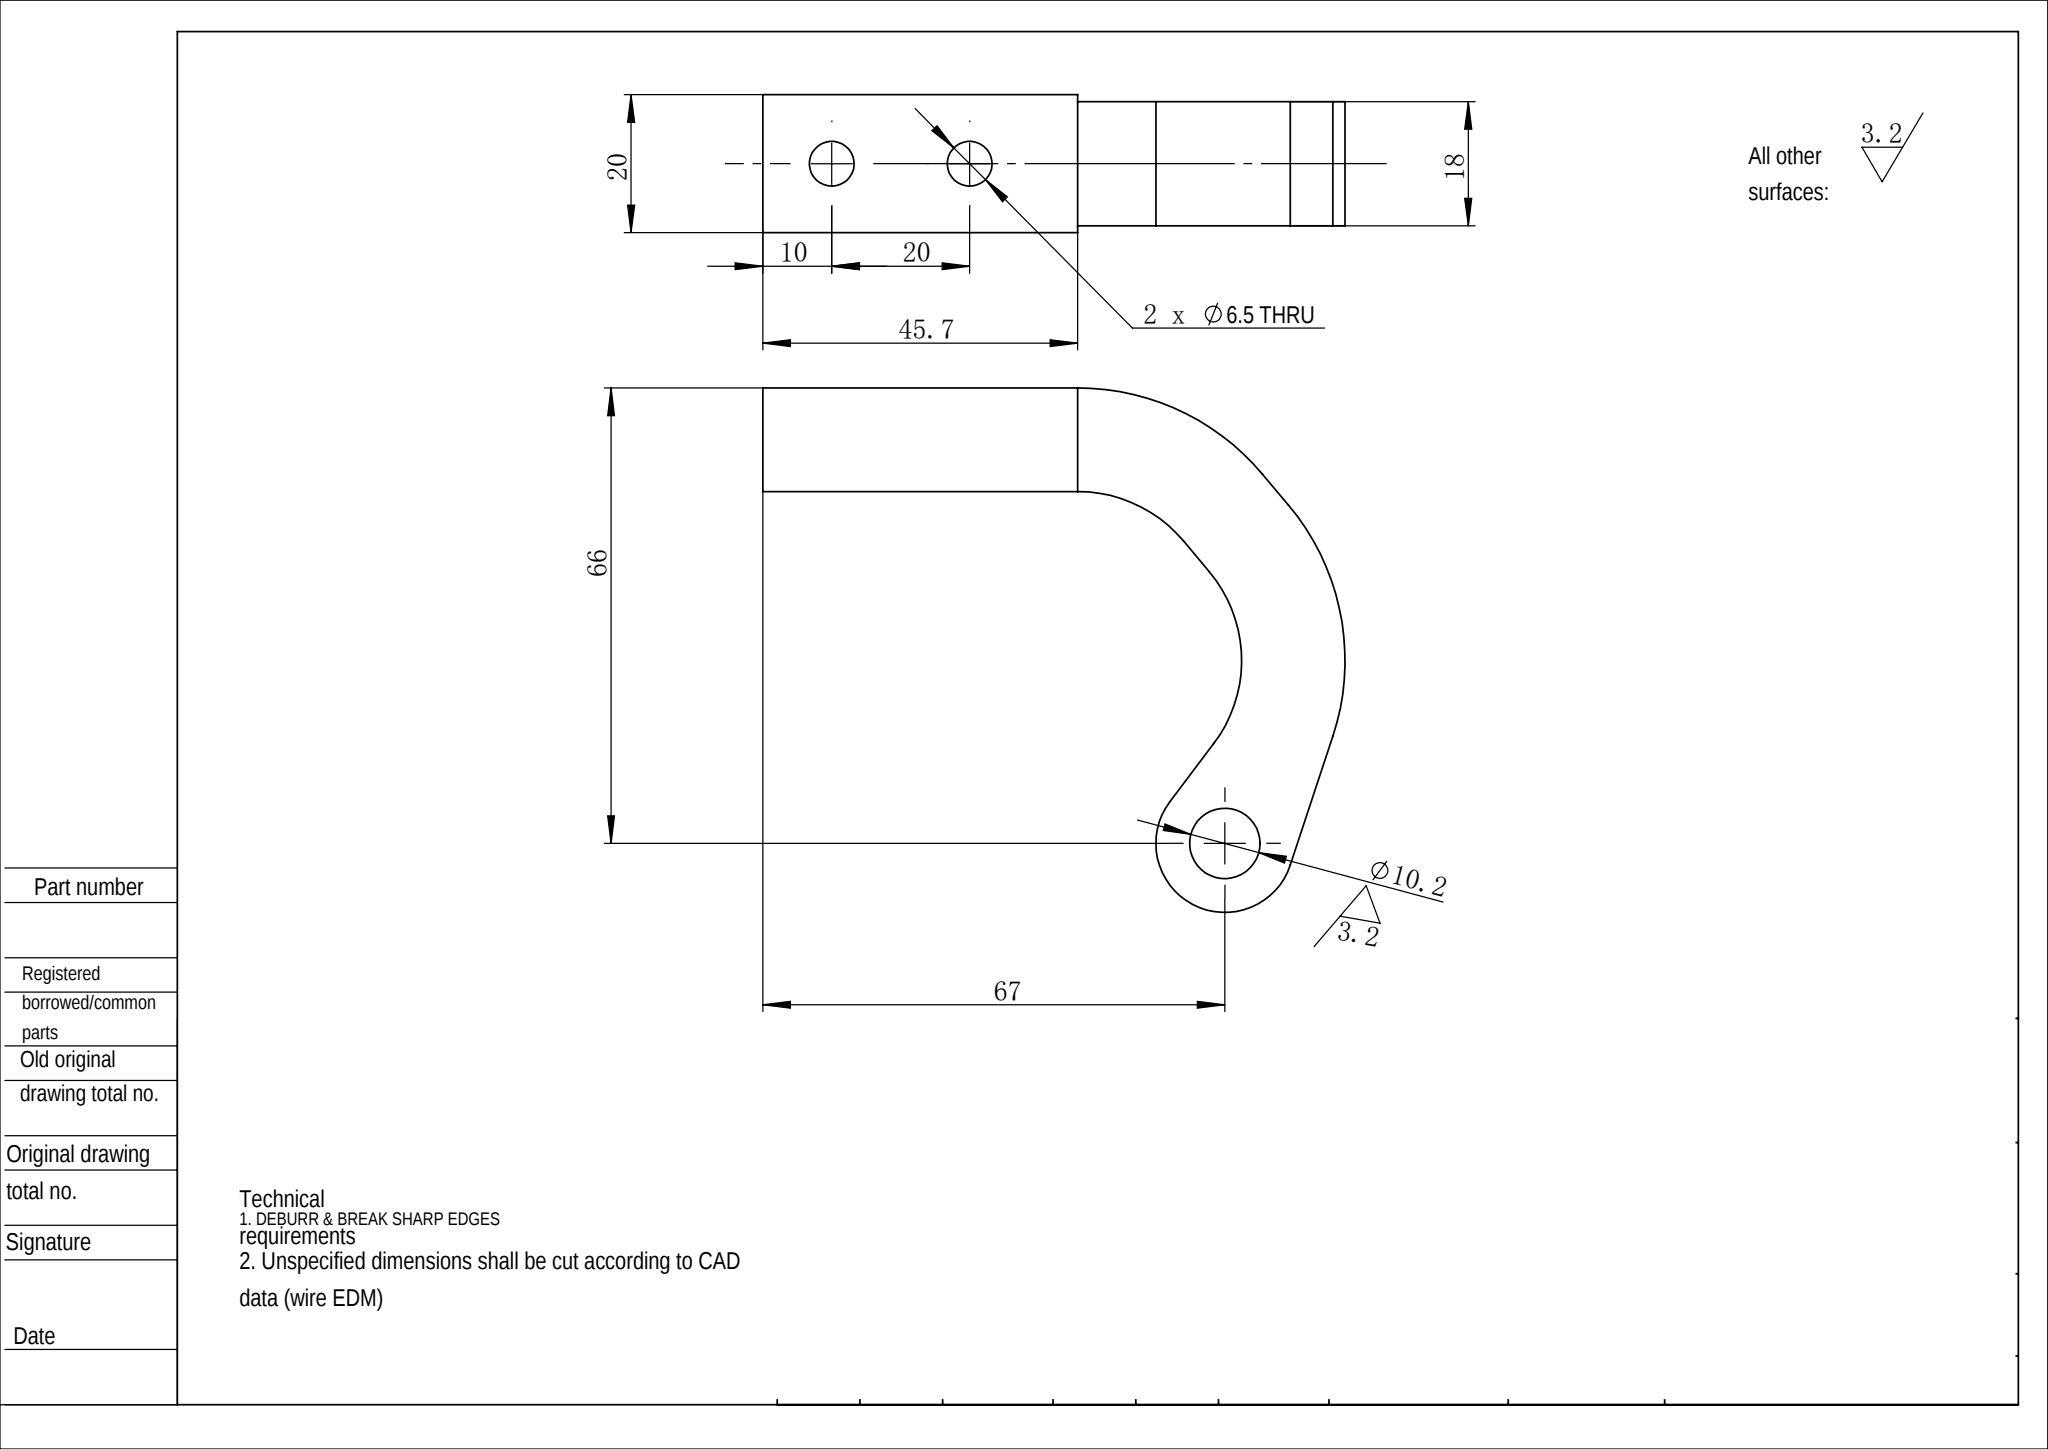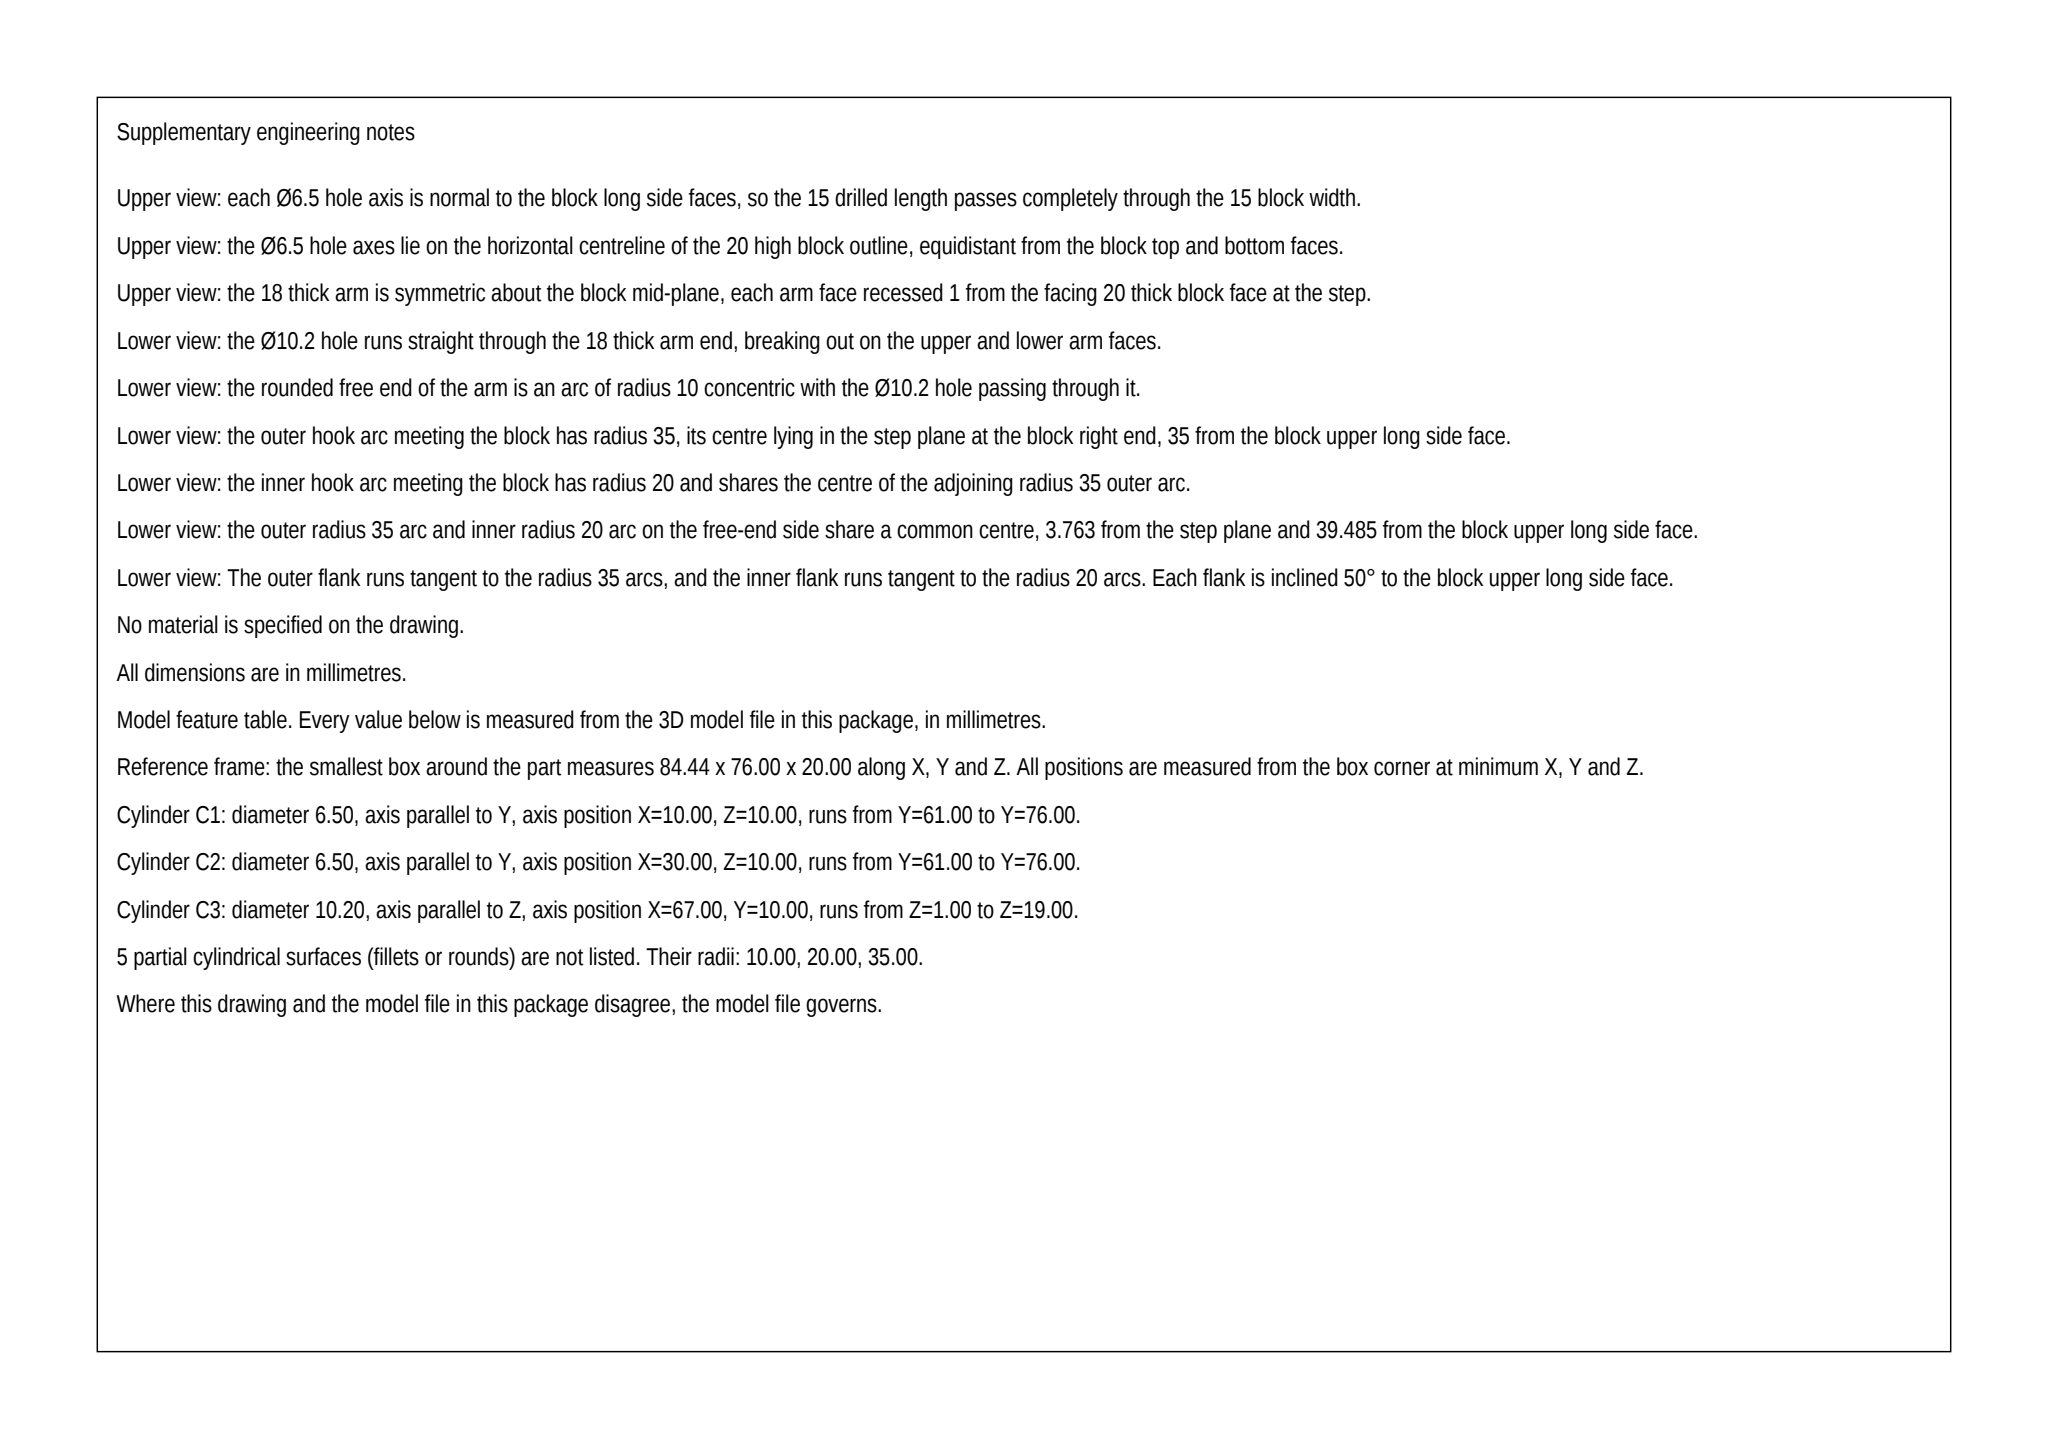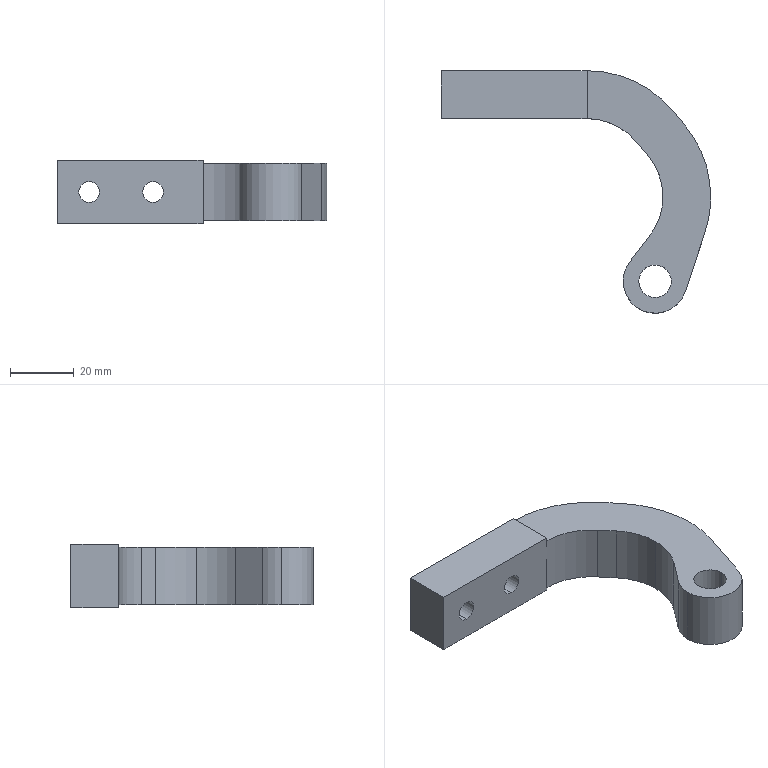Part | SolidWorks | mm | 1 solid | 27 faces | box 84.44 x 76 x 20 mm | volume 35805 mm3 | cylinder 14 | plane 13 | commonest cylinder face diameters 6.5 x4 70 x3 40 x3 10.2 x2 20 x2
Drawing notes:
OVERALL LG 84.44 FROM LH EDGE (TANGENT TO R35 OUTER ARC) | from the solid: bbox_xyz x = 84.437; outer R35 ctr x=49.44 + 35 = 84.44
ARM ARCS R20 INNER / R35 OUTER, CTR 45.67 FM LH EDGE, 35 BELOW TOP | from the solid: cylinders dia40 & dia70, axis z, pos (45.67, 41); top edge y=76, 76-41=35
ARM ARCS R20 INNER / R35 OUTER, CTR 49.44 FM LH EDGE, 39.48 BELOW TOP | from the solid: cylinders dia40 & dia70, axis z, pos (49.44, 36.52); 76-36.52=39.48
2 x Ø6.5 DP 15 FM TOP EDGE, BLIND - NOT THRU | from the solid: cylinders dia6.5 axis y, length 15, x=10 & 30, z=10, start at y=76
Ø20 BOSS CONC W/ Ø10.2 HOLE, 67 FM LH EDGE, 66 BELOW TOP | from the solid: cylinder dia20 axis z at (67,10) coincident with dia10.2 axis z at (67,10)
18 WIDE ARM CTRD ON 20 PLATE, 1 EA SIDE; STEP 45.67 FM LH EDGE | from the solid: z planes 0/1/19/20 (arm z=1..19 of 20); x planes at 45.67
FRONT VIEW PROFILE BREAK LINE 15 BELOW TOP EDGE | from the solid: axis plane y=61 vs top y=76; 76-61=15
build123d program:
from build123d import *
from build123d.topology import SkipClean

# Parameters (mm, degrees)
SKETCH1_R                      = 5.1
BOSS_EXTRUDE1_DEPTH            = 10
FILLET1_R                      = 20
CUT_EXTRUDE1_DEPTH             = 1
F_6_5_6_5_DIAMETER_HOLE1_D     = 6.5
F_6_5_6_5_DIAMETER_HOLE1_DEPTH = 15
F_6_5_6_5_DIAMETER_HOLE1_TIP   = 1.953
CUT_EXTRUDE2_DEPTH             = 188.122


with BuildPart() as part:
    # Sketch1 → Boss-Extrude1 (new body)
    with BuildSketch(Plane.XY):
        with BuildLine():
            Line((56.74, -38.548), (56.74, -53.548))
            Line((56.74, -53.548), (111.74, -53.548))
            Line((111.74, -53.548), (131.74, -77.383))
            Line((131.74, -77.383), (115.763, -98.517))
            ThreePointArc((115.763, -98.517), (114.787, -109.003), (123.74, -114.548))
            Line((123.74, -114.548), (146.74, -114.548))
            Line((146.74, -114.548), (146.74, -38.548))
            Line((146.74, -38.548), (56.74, -38.548))
        make_face()
        with Locations((123.74, -104.548)):
            Circle(SKETCH1_R, mode=Mode.SUBTRACT)
    extrude(amount=BOSS_EXTRUDE1_DEPTH)

    # Fillet1
    fillet1_edges = [part.edges().sort_by_distance(p)[0] for p in [
        (131.74, -77.383, 5),
        (111.74, -53.548, 5),
    ]]
    fillet(fillet1_edges, radius=FILLET1_R)

    # Sketch2 → Cut-Extrude1 (cut)
    with BuildSketch(Plane.XY.offset(10)):
        Polygon((102.414, -53.548), (102.414, -21.399), (217.212, -53.548), (217.212, -142.934), (102.414, -142.934), align=None)
    extrude(amount=-CUT_EXTRUDE1_DEPTH, mode=Mode.SUBTRACT)

    # Mirror1: part across plane


with BuildPart() as part_1:
    add(part.part)
    add(part.part.mirror(Plane(origin=(123.74, -104.548, 0), x_dir=(1, 0, 0), z_dir=(0, 0, 1))))

    # 6.5 _6.5_ Diameter Hole1
    with Locations(Plane(origin=(0, -53.548, 0), x_dir=(-1, 0, 0), z_dir=(0, -1, 0))):
        with Locations((-86.74, 0), (-66.74, 0)):
            Hole(F_6_5_6_5_DIAMETER_HOLE1_D / 2, depth=F_6_5_6_5_DIAMETER_HOLE1_DEPTH)
            with Locations((0, 0, -(F_6_5_6_5_DIAMETER_HOLE1_DEPTH + F_6_5_6_5_DIAMETER_HOLE1_TIP / 2))):  # 118° drill point
                Cone(0, F_6_5_6_5_DIAMETER_HOLE1_D / 2, F_6_5_6_5_DIAMETER_HOLE1_TIP, mode=Mode.SUBTRACT)

    # Sketch5 → Cut-Extrude2 (cut, through all)
    with SkipClean():  # the faces are left unmerged after this step: merging them gives an invalid solid
        with BuildSketch(Plane.XY.offset(9)):
            with BuildLine():
                Line((123.74, -114.548), (146.74, -114.548))
                Line((146.74, -114.548), (146.74, -38.548))
                Line((146.74, -38.548), (102.414, -38.548))
                ThreePointArc((102.414, -38.548), (117.205, -41.827), (129.225, -51.05))
                Line((129.225, -51.05), (132.988, -55.535))
                ThreePointArc((132.988, -55.535), (140.551, -71.444), (139.407, -89.022))
                Line((139.407, -89.022), (133.234, -107.688))
                ThreePointArc((133.234, -107.688), (129.596, -112.653), (123.74, -114.548))
            make_face()
        extrude(amount=-CUT_EXTRUDE2_DEPTH, mode=Mode.SUBTRACT)


solid = part_1.part